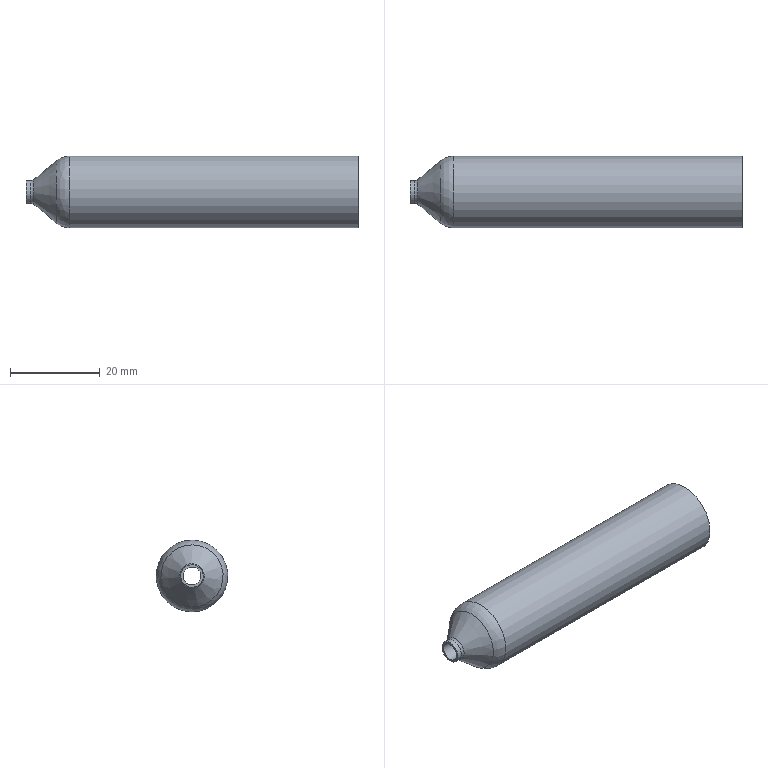Component | NX | LUMEN | 1 solid | 10 faces | volume 5193 mm3 | cylinder 4 | plane 2 | spline 2 | cone 1 | torus 1 | commonest cylinder face diameters 16 x1 5 x1 13 x1 4 x1